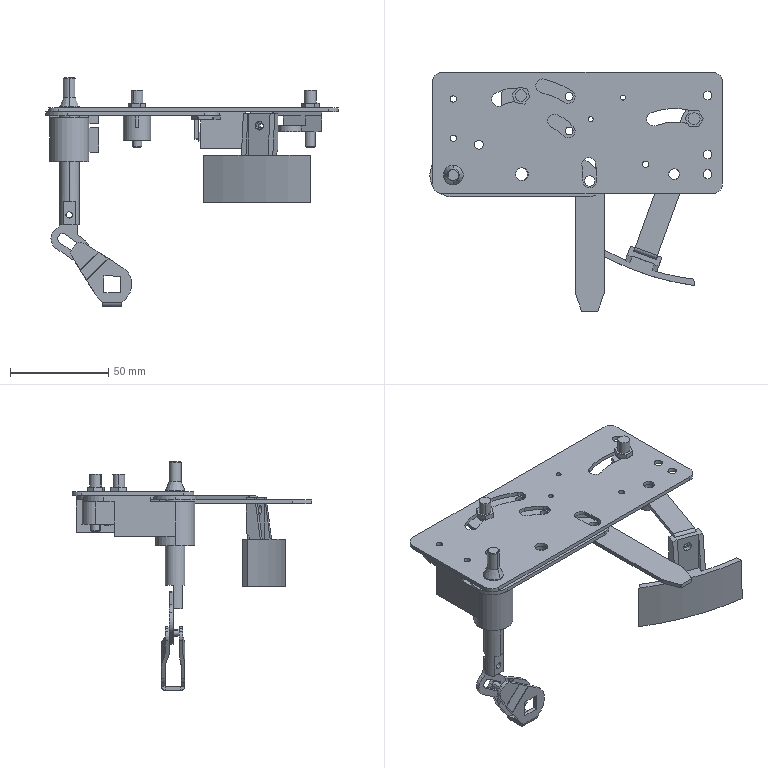Assembly | SolidWorks | mm | 14 component files | 14 solids | 378 faces | box 149 x 122.2 x 116.62 mm | volume 72004 mm3 | plane 189 | cylinder 179 | cone 8 | torus 2 | commonest cylinder face diameters 5.5 x18 3.2 x14 7 x14 6 x14 4.5 x12 10 x10 20 x9 1 x8
Bill of materials:
CLS-MechanismAccessory1 | 1 |  | Elongated block-like part with a tall cylindrical boss at one end containing a large through bore, a raised flat arm with an obround end carrying two smaller through holes, and two thin parallel fins projecting from one side.
CLS-MechanismAccessory2 | 1 |  | Stadium-shaped (obround) solid block with a round through hole near one end and a narrow straight slot running from that hole out to the opposite rounded end, making a keyhole-like opening from the top.
CLS-MechanismAccessory3 | 1 |  | Flat obround link bar with a round hole at each rounded end. One end is a thinner lug, and the rest of the bar is a thicker raised section, which forms a step.
CLS-MechanismAccessory4 | 1 | 2.0 Galvanized Sheet Q235A | L-shaped bent strip bracket: a long flat arm with a rounded end and two round holes, bent 90 degrees at a radiused corner into a short leg with a square-cut end and two round holes of different sizes.
CLS-MechanismAccessory5 | 2 | 10 Cold Drawn Round Steel GB699-88 | Cylindrical pin with a hexagonal collar near one end: a short cylindrical section above the hex, and a longer, slightly smaller shank below with a chamfered tip.
CLS-MechanismAuxiliarySwitch | 1 | 2.0 Galvanized Sheet Q235A | Rectangular block with two round through holes on the top face at diagonally opposite positions, plus a small rectangular projection on one side face.
CLS-MechanismBasePlate | 1 | 2.0 Galvanized Sheet Q235A | Thin flat rectangular plate with rounded corners, pierced by many round holes of several sizes and several curved arc-shaped slots plus one nearly straight slot.
CLS-MechanismIndicatorPlate | 1 |  | Curved band segment (part of a ring) with a perpendicular upright tab rising from its middle. The tab has notched edges, a round through hole near its top and a small cylindrical pin or boss.
CLS-MechanismLimitSwitchStopPlate | 1 | 2.0 Galvanized Sheet Q235A | Flat sheet-style plate with an irregular L-like outline and rounded corners. It has a large hole in one rounded lobe, several smaller round holes, and a flange bent down 90 degrees along one edge, with relief notches at both ends of the bend.
CLS-MechanismOperatingAxisBracket | 1 |  | U-shaped bent strap clevis form: two tapered side plates joined by a curved bend at one end, and a cylindrical spacer bridging them at the other end. Aligned square holes pass through both side plates.
CLS-MechanismPositioningPin | 1 | 10 Cold Drawn Round Steel GB699-88 | Stepped cylindrical shaft: a reduced-diameter end section joined to the main body by a conical taper. The opposite end is machined with a flat and has a small cross hole through it.
CLS-MechanismPositioningSlide | 1 |  | Flat plate tab of constant thickness: a rectangular upper tongue with a round hole, blending through a curved fillet into a rounded lower lobe that has an angled elongated slot.
CLS-MechanismTopPlate | 1 | 2.0 Galvanized Sheet Q235A | Thin, flat, elongated plate of uniform thickness. One end is a full semicircle with a single round through-hole near it. The other end tapers symmetrically with two angled edges to a narrower flat tip.
Mates:
1. concentric | CLS-MechanismBasePlate-1 edge at (-59.026, 15.442, -3.001) dir (0, 0, 1) r 1.6 | CLS-MechanismAccessory1-1 edge at (-59.026, 15.442, -6.001) dir (0, 0, -1) r 2.75
2. coincident | CLS-MechanismBasePlate-1 face at (72.974, 24.192, -3.001) dir (0, 0, -1) | CLS-MechanismAccessory1-1 face at (-69.026, 23.192, -3.001) dir (0, 0, 1)
3. parallel | CLS-MechanismBasePlate-1 face at (-69.526, 24.192, -3.001) dir (-1, 0, 0) | CLS-MechanismAccessory1-1 face at (-69.026, -33.308, -23.501) dir (-1, 0, 0)
4. concentric | CLS-MechanismBasePlate-1 edge at (-59.026, -23.308, -1.001) dir (0, 0, 1) r 5 | CLS-MechanismLimitSwitchStopPlate-1 edge at (-59.026, -23.308, -5.001) dir (0, 0, -1) r 6.25
5. coincident | CLS-MechanismBasePlate-1 face at (72.974, 24.192, -3.001) dir (0, 0, -1) | CLS-MechanismLimitSwitchStopPlate-1 face at (-71.026, -34.308, -3.001) dir (0, 0, 1)
6. parallel | CLS-MechanismBasePlate-1 face at (-64.526, -32.808, -3.001) dir (0, -1, 0) | CLS-MechanismLimitSwitchStopPlate-1 face at (17.474, -34.308, -3.001) dir (0, -1, 0)
7. concentric | CLS-MechanismAccessory2-1 edge at (-24.526, 17.192, -17.501) dir (0, 0, -1) r 2.75 | CLS-MechanismLimitSwitchStopPlate-1 edge at (-24.526, 17.192, -5.001) dir (0, 0, -1) r 2.75
8. coincident | CLS-MechanismAccessory2-1 face at (-24.526, 17.192, -5.001) dir (0, 0, 1) | CLS-MechanismLimitSwitchStopPlate-1 face at (-71.026, -34.308, -5.001) dir (0, 0, -1)
9. parallel | CLS-MechanismAccessory2-1 face at (-31.526, 17.192, -17.501) dir (-1, 0, 0) | CLS-MechanismLimitSwitchStopPlate-1 face at (-34.526, 26.692, -3.001) dir (-1, 0, 0)
10. concentric | CLS-MechanismBasePlate-1 edge at (53.474, -22.808, -3.001) dir (0, 0, 1) r 2.75 | CLS-MechanismAccessory3-1 edge at (53.474, -22.808, -13.001) dir (0, 0, -1) r 2.75
11. distance | CLS-MechanismBasePlate-1 face at (72.974, 24.192, -3.001) dir (0, 0, -1) | CLS-MechanismAccessory3-1 face at (63.64, 5.417, -5.001) dir (0, 0, 1)
12. concentric | CLS-MechanismLimitSwitchStopPlate-1 edge at (10.474, -26.308, -5.001) dir (0, 0, -1) r 2.6 | CLS-MechanismTopPlate-1 edge at (10.474, -26.308, -7.001) dir (0, 0, -1) r 2.6
13. coincident | CLS-MechanismLimitSwitchStopPlate-1 face at (-71.026, -34.308, -5.001) dir (0, 0, -1) | CLS-MechanismTopPlate-1 face at (2.974, -93.008, -5.001) dir (0, 0, 1)
14. concentric | CLS-MechanismAccessory4-1 edge at (63.64, 5.417, -5.001) dir (0, 0, 1) r 2.75 | CLS-MechanismAccessory3-1 edge at (63.64, 5.417, -13.001) dir (0, 0, -1) r 2.75
15. parallel | CLS-MechanismAccessory4-1 face at (60.029, 13.095, -5.001) dir (-0.9408, 0.3389, 0) | CLS-MechanismAccessory3-1 face at (57.995, 7.45, -13.001) dir (-0.9408, 0.3389, 0)
16. concentric | CLS-MechanismAccessory4-1 edge at (38.563, -64.204, -10.001) dir (-0.3389, -0.9408, 0) r 1.25 | CLS-MechanismIndicatorPlate-1 edge at (37.715, -66.556, -10.001) dir (0.3389, 0.9408, 0) r 2.25
17. coincident | CLS-MechanismAccessory4-1 face at (32.918, -62.171, -5.001) dir (-0.3389, -0.9408, 0) | CLS-MechanismIndicatorPlate-1 face at (12.69, -54.885, -25.001) dir (0.3389, 0.9408, 0)
18. parallel | CLS-MechanismAccessory4-1 face at (32.918, -62.171, -26.001) dir (-0.9408, 0.3389, 0) | CLS-MechanismIndicatorPlate-1 face at (29.583, -64.052, -25.001) dir (-0.9408, 0.3389, 0)
19. concentric | CLS-MechanismAccessory3-1 edge at (63.64, 5.417, -13.001) dir (0, 0, -1) r 2.75 | CLS-MechanismAccessory5-1 edge at (63.64, 5.417, 7.999) dir (0, 0, 1) r 3
20. coincident | CLS-MechanismBasePlate-1 face at (72.974, 24.192, -1.001) dir (0, 0, 1) | CLS-MechanismAccessory5-1 face at (65.95, 1.417, -1.001) dir (0, 0, -1)
21. concentric | CLS-MechanismAccessory2-1 edge at (-24.526, 17.192, -17.501) dir (0, 0, -1) r 2.75 | CLS-MechanismAccessory5-2 edge at (-24.526, 17.192, 7.999) dir (0, 0, 1) r 3
22. coincident | CLS-MechanismBasePlate-1 face at (72.974, 24.192, -1.001) dir (0, 0, 1) | CLS-MechanismAccessory5-2 face at (-19.989, 16.329, -1.001) dir (0, 0, -1)
23. parallel | CLS-MechanismBasePlate-1 face at (77.974, 24.192, -3.001) dir (1, 0, 0) | CLS-MechanismTopPlate-1 face at (17.974, -18.808, -7.001) dir (1, 0, 0)
24. concentric | CLS-MechanismBasePlate-1 edge at (27.474, 16.192, -3.001) dir (0, 0, 1) r 1.25 | CLS-MechanismAuxiliarySwitch-1 edge at (27.474, 16.192, -21.501) dir (0, 0, -1) r 1.6
25. coincident | CLS-MechanismBasePlate-1 face at (72.974, 24.192, -3.001) dir (0, 0, -1) | CLS-MechanismAuxiliarySwitch-1 face at (7.974, -4.449, -3.001) dir (0, 0, 1)
26. parallel | CLS-MechanismBasePlate-1 face at (77.974, 24.192, -3.001) dir (1, 0, 0) | CLS-MechanismAuxiliarySwitch-1 face at (30.474, 27.051, -3.001) dir (1, 0, 0)
27. coincident | CLS-MechanismAccessory4-1 face at (32.918, -62.171, -5.001) dir (0, 0, -1) | CLS-MechanismAccessory3-1 face at (63.64, 5.417, -5.001) dir (0, 0, 1)
28. concentric | CLS-MechanismAccessory1-1 edge at (-59.026, -23.308, -28.501) dir (0, 0, -1) r 6.5 | CLS-MechanismOperatingAxisBracketAssembly.SLDPRT-1/CLS-MechanismPositioningPin-1 edge at (-59.026, -23.308, 14.209) dir (0, 0, -1) r 3
29. parallel | CLS-MechanismLimitSwitchStopPlate-1 face at (17.474, -34.308, -3.001) dir (0, -1, 0) | CLS-MechanismOperatingAxisBracketAssembly.SLDPRT-1/CLS-MechanismPositioningPin-1 face at (-59.026, -27.308, -48.491) dir (0, -1, 0)
30. concentric | CLS-MechanismPositioningPin-1 edge at (19.895, 7.201, 17.42) dir (0, 1, 0) r 1.6 | CLS-MechanismPositioningSlide-1 edge at (19.895, 0.2013, 17.42) dir (0, -1, 0) r 1.6
31. coincident | CLS-MechanismPositioningPin-1 face at (19.794, 2.201, 24.42) dir (0, -1, 0) | CLS-MechanismPositioningSlide-1 face at (15.837, 2.201, 0.2116) dir (0, 1, 0)
32. parallel | CLS-MechanismPositioningPin-1 face at (19.794, 3.201, 12.42) dir (0, 0, -1) | CLS-MechanismPositioningSlide-1 face at (24.145, 2.201, 21.42) dir (0, 0, 1)
33. distance | CLS-MechanismOperatingAxisBracket-1 face at (24.356, 0.2013, -5.394) dir (0, 1, 0) | CLS-MechanismPositioningSlide-1 face at (15.837, 2.201, 0.2116) dir (0, 1, 0)
34. parallel | CLS-MechanismPositioningPin-1 face at (19.794, 3.201, 12.42) dir (0, 0, -1) | CLS-MechanismPositioningSlide-1 axis at (23.19, 2.201, 5.402) dir (0, -1, 0)
35. parallel | CLS-MechanismPositioningPin-1 face at (19.794, 3.201, 12.42) dir (0, 0, -1) | CLS-MechanismOperatingAxisBracketAssembly.SLDPRT plane at (0, 0, 0) dir (0, 0, 1)
36. concentric | CLS-MechanismOperatingAxisBracket-1 edge at (15.837, 5.201, 0.2116) dir (0, 1, 0) r 1.75 | CLS-MechanismPositioningSlide-1 edge at (15.837, 2.201, 0.2116) dir (0, -1, 0) r 2.5